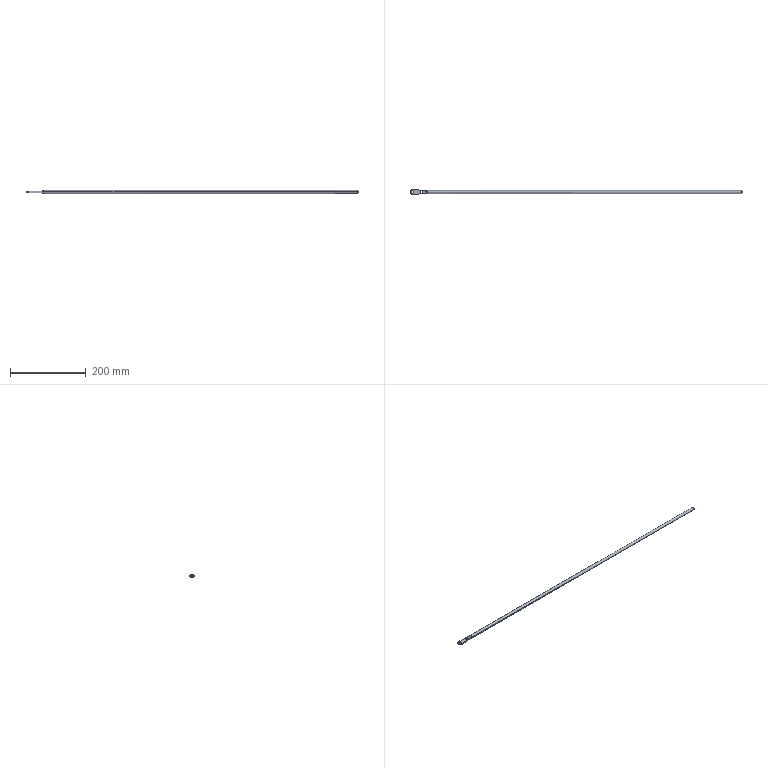Component | SolidWorks | RightRearDoorFrameAssembly-1_RearDoorLowerLockRod-1 | 1 solid | 20 faces | box 878.5 x 13 x 8 mm | volume 43100 mm3 | plane 11 | cylinder 7 | cone 2 | commonest cylinder face diameters 6.5 x4 8 x2 13 x1
build123d program:
from build123d import *

# Parameters (mm, degrees)
SKETCH1_R           = 4
BOSS_EXTRUDE1_DEPTH = 878.5
CUT_EXTRUDE1_DEPTH  = 5
SKETCH3_W           = 42
SKETCH3_H           = 2.024
CUT_EXTRUDE2_DEPTH  = 10
BOSS_EXTRUDE2_DEPTH = 3
CUT_EXTRUDE3_DEPTH  = 3
SKETCH6_R           = 3.25
CUT_EXTRUDE4_DEPTH  = 3
CHAMFER1_SIZE       = 1.5


with BuildPart() as part:
    # Sketch1 → Boss-Extrude1 (new body)
    with BuildSketch(Plane(origin=(0, 0, 0), x_dir=(0, 0, -1), z_dir=(1, 0, 0))):
        Circle(SKETCH1_R)
    extrude(amount=-BOSS_EXTRUDE1_DEPTH)

    # Sketch2 → Cut-Extrude1 (cut, symmetric)
    with BuildSketch(Plane.XY):
        Polygon((-42, 1.5), (-45.678, 4), (-42, 4), (0, 4), (0, 1.5), align=None)
        Polygon((-45.678, -4), (-42, -4), (0, -4), (0, -1.5), (-42, -1.5), align=None)
    extrude(amount=CUT_EXTRUDE1_DEPTH, both=True, mode=Mode.SUBTRACT)

    # Sketch3 → Cut-Extrude2 (cut)
    with BuildSketch(Plane(origin=(0, 1.5, 0), x_dir=(1, 0, 0), z_dir=(0, 1, 0))):
        with Locations((-21, 2.988)):
            Rectangle(SKETCH3_W, SKETCH3_H)
        with Locations((-21, -2.988)):
            Rectangle(SKETCH3_W, SKETCH3_H)
    extrude(amount=-CUT_EXTRUDE2_DEPTH, mode=Mode.SUBTRACT)

    # Sketch4 → Boss-Extrude2 (add)
    with BuildSketch(Plane(origin=(0, 1.5, 0), x_dir=(1, 0, 0), z_dir=(0, 1, 0))):
        with BuildLine():
            Line((-42, -4), (-42, 4))
            Line((-42, 4), (-7.386, 6.439))
            ThreePointArc((-7.386, 6.439), (0, 0), (-7.386, -6.439))
            Line((-7.386, -6.439), (-42, -4))
        make_face()
    extrude(amount=-BOSS_EXTRUDE2_DEPTH)

    # Sketch5 → Cut-Extrude3 (cut)
    with BuildSketch(Plane(origin=(0, 1.5, 0), x_dir=(1, 0, 0), z_dir=(0, 1, 0))):
        with BuildLine():
            Line((-0.8017, 3.127), (2.344, 3.127))
            Line((2.344, 3.127), (2.344, -3.404))
            Line((2.344, -3.404), (-0.9628, -3.404))
            ThreePointArc((-0.9628, -3.404), (-0.001977, -0.1603), (-0.8017, 3.127))
        make_face()
    extrude(amount=-CUT_EXTRUDE3_DEPTH, mode=Mode.SUBTRACT)

    # Sketch6 → Cut-Extrude4 (cut)
    with BuildSketch(Plane(origin=(0, 1.5, 0), x_dir=(1, 0, 0), z_dir=(0, 1, 0))):
        with Locations(Location((-6, 0, 0), (0, 0, 180))):
            Circle(SKETCH6_R)
        with Locations(Location((-31, 0, 0), (0, 0, 180))):
            Circle(SKETCH6_R)
    extrude(amount=-CUT_EXTRUDE4_DEPTH, mode=Mode.SUBTRACT)

    # Chamfer1
    chamfer1_edges = [part.edges().sort_by_distance(p)[0] for p in [
        (-878.5, 0, 4),
    ]]
    chamfer(chamfer1_edges, length=CHAMFER1_SIZE)


solid = part.part

# Placed as in the assembly
solid = solid.moved(Location((30.814, 303.707, -28.746), (-90, 0, 180)))
STEP:
#1=COLOUR_RGB('',0.7922,0.8196,0.9333);
#2=FILL_AREA_STYLE_COLOUR('',#1);
#3=FILL_AREA_STYLE('',(#2));
#4=SURFACE_STYLE_FILL_AREA(#3);
#5=SURFACE_SIDE_STYLE('',(#4));
#6=SURFACE_STYLE_USAGE(.BOTH.,#5);
#7=PRESENTATION_STYLE_ASSIGNMENT((#6));
#8=CARTESIAN_POINT('',(35.8,12.055,-1.132));
#9=VERTEX_POINT('',#8);
#10=CARTESIAN_POINT('',(35.8,11.859,-1.132));
#11=VERTEX_POINT('',#10);
#12=CARTESIAN_POINT('',(35.8,11.957,-1.132));
#13=DIRECTION('',(1.,-0.,0.));
#14=DIRECTION('',(0.,-1.,0.));
#15=AXIS2_PLACEMENT_3D('',#12,#13,#14);
#16=CIRCLE('',#15,0.09843);
#17=EDGE_CURVE('',#9,#11,#16,.T.);
#18=ORIENTED_EDGE('',*,*,#17,.F.);
#19=CARTESIAN_POINT('',(35.741,12.114,-1.132));
#20=VERTEX_POINT('',#19);
#21=CARTESIAN_POINT('',(35.741,12.114,-1.132));
#22=DIRECTION('',(-0.7071,0.7071,-0.));
#23=VECTOR('',#22,39.37);
#24=LINE('',#21,#23);
#25=EDGE_CURVE('',#9,#20,#24,.T.);
#26=ORIENTED_EDGE('',*,*,#25,.T.);
#27=CARTESIAN_POINT('',(35.741,11.799,-1.132));
#28=VERTEX_POINT('',#27);
#29=CARTESIAN_POINT('',(35.741,11.957,-1.132));
#30=DIRECTION('',(-1.,0.,-0.));
#31=DIRECTION('',(0.,-1.,0.));
#32=AXIS2_PLACEMENT_3D('',#29,#30,#31);
#33=CIRCLE('',#32,0.1575);
#34=EDGE_CURVE('',#28,#20,#33,.T.);
#35=ORIENTED_EDGE('',*,*,#34,.F.);
#36=CARTESIAN_POINT('',(35.741,11.799,-1.132));
#37=DIRECTION('',(-0.7071,-0.7071,-0.));
#38=VECTOR('',#37,39.37);
#39=LINE('',#36,#38);
#40=EDGE_CURVE('',#11,#28,#39,.T.);
#41=ORIENTED_EDGE('',*,*,#40,.F.);
#42=EDGE_LOOP('',(#18,#26,#35,#41));
#43=FACE_OUTER_BOUND('',#42,.T.);
#44=CARTESIAN_POINT('',(35.741,11.957,-1.132));
#45=DIRECTION('',(-1.,0.,-0.));
#46=DIRECTION('',(0.,-1.,0.));
#47=AXIS2_PLACEMENT_3D('',#44,#45,#46);
#48=CONICAL_SURFACE('',#47,0.1575,0.7854);
#49=ADVANCED_FACE('',(#43),#48,.T.);
#50=CARTESIAN_POINT('',(2.306,11.957,-1.191));
#51=VERTEX_POINT('',#50);
#52=CARTESIAN_POINT('',(2.562,11.957,-1.191));
#53=VERTEX_POINT('',#52);
#54=CARTESIAN_POINT('',(2.434,11.957,-1.191));
#55=DIRECTION('',(-0.,-0.,1.));
#56=DIRECTION('',(1.,0.,0.));
#57=AXIS2_PLACEMENT_3D('',#54,#55,#56);
#58=CIRCLE('',#57,0.128);
#59=EDGE_CURVE('',#51,#53,#58,.T.);
#60=ORIENTED_EDGE('',*,*,#59,.F.);
#61=CARTESIAN_POINT('',(2.306,11.957,-1.073));
#62=VERTEX_POINT('',#61);
#63=CARTESIAN_POINT('',(2.306,11.957,-1.191));
#64=DIRECTION('',(-0.,-0.,1.));
#65=VECTOR('',#64,39.37);
#66=LINE('',#63,#65);
#67=EDGE_CURVE('',#51,#62,#66,.T.);
#68=ORIENTED_EDGE('',*,*,#67,.T.);
#69=CARTESIAN_POINT('',(2.562,11.957,-1.073));
#70=VERTEX_POINT('',#69);
#71=CARTESIAN_POINT('',(2.434,11.957,-1.073));
#72=DIRECTION('',(-0.,-0.,1.));
#73=DIRECTION('',(1.,0.,0.));
#74=AXIS2_PLACEMENT_3D('',#71,#72,#73);
#75=CIRCLE('',#74,0.128);
#76=EDGE_CURVE('',#62,#70,#75,.T.);
#77=ORIENTED_EDGE('',*,*,#76,.T.);
#78=CARTESIAN_POINT('',(2.562,11.957,-1.191));
#79=DIRECTION('',(-0.,-0.,1.));
#80=VECTOR('',#79,39.37);
#81=LINE('',#78,#80);
#82=EDGE_CURVE('',#53,#70,#81,.T.);
#83=ORIENTED_EDGE('',*,*,#82,.F.);
#84=EDGE_LOOP('',(#60,#68,#77,#83));
#85=FACE_OUTER_BOUND('',#84,.T.);
#86=CARTESIAN_POINT('',(2.434,11.957,-1.191));
#87=DIRECTION('',(-0.,-0.,1.));
#88=DIRECTION('',(1.,0.,0.));
#89=AXIS2_PLACEMENT_3D('',#86,#87,#88);
#90=CYLINDRICAL_SURFACE('',#89,0.128);
#91=ADVANCED_FACE('',(#85),#90,.F.);
#92=CARTESIAN_POINT('',(1.321,11.957,-1.191));
#93=VERTEX_POINT('',#92);
#94=CARTESIAN_POINT('',(1.577,11.957,-1.191));
#95=VERTEX_POINT('',#94);
#96=CARTESIAN_POINT('',(1.449,11.957,-1.191));
#97=DIRECTION('',(-0.,-0.,1.));
#98=DIRECTION('',(1.,0.,0.));
#99=AXIS2_PLACEMENT_3D('',#96,#97,#98);
#100=CIRCLE('',#99,0.128);
#101=EDGE_CURVE('',#93,#95,#100,.T.);
#102=ORIENTED_EDGE('',*,*,#101,.F.);
#103=CARTESIAN_POINT('',(1.321,11.957,-1.073));
#104=VERTEX_POINT('',#103);
#105=CARTESIAN_POINT('',(1.321,11.957,-1.191));
#106=DIRECTION('',(-0.,-0.,1.));
#107=VECTOR('',#106,39.37);
#108=LINE('',#105,#107);
#109=EDGE_CURVE('',#93,#104,#108,.T.);
#110=ORIENTED_EDGE('',*,*,#109,.T.);
#111=CARTESIAN_POINT('',(1.577,11.957,-1.073));
#112=VERTEX_POINT('',#111);
#113=CARTESIAN_POINT('',(1.449,11.957,-1.073));
#114=DIRECTION('',(-0.,-0.,1.));
#115=DIRECTION('',(1.,0.,0.));
#116=AXIS2_PLACEMENT_3D('',#113,#114,#115);
#117=CIRCLE('',#116,0.128);
#118=EDGE_CURVE('',#104,#112,#117,.T.);
#119=ORIENTED_EDGE('',*,*,#118,.T.);
#120=CARTESIAN_POINT('',(1.577,11.957,-1.191));
#121=DIRECTION('',(-0.,-0.,1.));
#122=VECTOR('',#121,39.37);
#123=LINE('',#120,#122);
#124=EDGE_CURVE('',#95,#112,#123,.T.);
#125=ORIENTED_EDGE('',*,*,#124,.F.);
#126=EDGE_LOOP('',(#102,#110,#119,#125));
#127=FACE_OUTER_BOUND('',#126,.T.);
#128=CARTESIAN_POINT('',(1.449,11.957,-1.191));
#129=DIRECTION('',(-0.,-0.,1.));
#130=DIRECTION('',(1.,0.,0.));
#131=AXIS2_PLACEMENT_3D('',#128,#129,#130);
#132=CYLINDRICAL_SURFACE('',#131,0.128);
#133=ADVANCED_FACE('',(#127),#132,.F.);
#134=ORIENTED_EDGE('',*,*,#34,.T.);
#135=CARTESIAN_POINT('',(2.867,12.114,-1.132));
#136=VERTEX_POINT('',#135);
#137=CARTESIAN_POINT('',(35.8,12.114,-1.132));
#138=DIRECTION('',(-1.,0.,-0.));
#139=VECTOR('',#138,39.37);
#140=LINE('',#137,#139);
#141=EDGE_CURVE('',#20,#136,#140,.T.);
#142=ORIENTED_EDGE('',*,*,#141,.T.);
#143=CARTESIAN_POINT('',(2.867,12.103,-1.073));
#144=VERTEX_POINT('',#143);
#145=CARTESIAN_POINT('',(2.867,11.957,-1.132));
#146=DIRECTION('',(-1.,0.,-0.));
#147=DIRECTION('',(0.,-0.,-1.));
#148=AXIS2_PLACEMENT_3D('',#145,#146,#147);
#149=CIRCLE('',#148,0.1575);
#150=EDGE_CURVE('',#144,#136,#149,.T.);
#151=ORIENTED_EDGE('',*,*,#150,.F.);
#152=CARTESIAN_POINT('',(2.867,11.811,-1.073));
#153=VERTEX_POINT('',#152);
#154=CARTESIAN_POINT('',(2.867,11.811,-1.073));
#155=CARTESIAN_POINT('',(3.094,11.874,-0.918));
#156=CARTESIAN_POINT('',(3.094,12.04,-0.918));
#157=CARTESIAN_POINT('',(2.867,12.103,-1.073));
#158=(BOUNDED_CURVE()B_SPLINE_CURVE(3,(#154,#155,#156,#157),.UNSPECIFIED.,.F.,.F.)B_SPLINE_CURVE_WITH_KNOTS((4,4),(1.955,4.328),.UNSPECIFIED.)CURVE()GEOMETRIC_REPRESENTATION_ITEM()RATIONAL_B_SPLINE_CURVE((1.,0.5833,0.5833,1.))REPRESENTATION_ITEM(''));
#159=EDGE_CURVE('',#153,#144,#158,.T.);
#160=ORIENTED_EDGE('',*,*,#159,.F.);
#161=CARTESIAN_POINT('',(2.867,11.799,-1.132));
#162=VERTEX_POINT('',#161);
#163=CARTESIAN_POINT('',(2.867,11.957,-1.132));
#164=DIRECTION('',(-1.,0.,-0.));
#165=DIRECTION('',(0.,-0.,-1.));
#166=AXIS2_PLACEMENT_3D('',#163,#164,#165);
#167=CIRCLE('',#166,0.1575);
#168=EDGE_CURVE('',#162,#153,#167,.T.);
#169=ORIENTED_EDGE('',*,*,#168,.F.);
#170=CARTESIAN_POINT('',(35.8,11.799,-1.132));
#171=DIRECTION('',(-1.,0.,-0.));
#172=VECTOR('',#171,39.37);
#173=LINE('',#170,#172);
#174=EDGE_CURVE('',#28,#162,#173,.T.);
#175=ORIENTED_EDGE('',*,*,#174,.F.);
#176=EDGE_LOOP('',(#134,#142,#151,#160,#169,#175));
#177=FACE_OUTER_BOUND('',#176,.T.);
#178=CARTESIAN_POINT('',(35.8,11.957,-1.132));
#179=DIRECTION('',(-1.,0.,-0.));
#180=DIRECTION('',(0.,-1.,0.));
#181=AXIS2_PLACEMENT_3D('',#178,#179,#180);
#182=CYLINDRICAL_SURFACE('',#181,0.1575);
#183=ADVANCED_FACE('',(#177),#182,.T.);
#184=ORIENTED_EDGE('',*,*,#141,.F.);
#185=CARTESIAN_POINT('',(35.741,11.957,-1.132));
#186=DIRECTION('',(-1.,0.,-0.));
#187=DIRECTION('',(0.,-1.,0.));
#188=AXIS2_PLACEMENT_3D('',#185,#186,#187);
#189=CIRCLE('',#188,0.1575);
#190=EDGE_CURVE('',#20,#28,#189,.T.);
#191=ORIENTED_EDGE('',*,*,#190,.T.);
#192=ORIENTED_EDGE('',*,*,#174,.T.);
#193=CARTESIAN_POINT('',(2.867,11.811,-1.191));
#194=VERTEX_POINT('',#193);
#195=CARTESIAN_POINT('',(2.867,11.957,-1.132));
#196=DIRECTION('',(-1.,0.,-0.));
#197=DIRECTION('',(0.,-0.,-1.));
#198=AXIS2_PLACEMENT_3D('',#195,#196,#197);
#199=CIRCLE('',#198,0.1575);
#200=EDGE_CURVE('',#194,#162,#199,.T.);
#201=ORIENTED_EDGE('',*,*,#200,.F.);
#202=CARTESIAN_POINT('',(2.867,12.103,-1.191));
#203=VERTEX_POINT('',#202);
#204=CARTESIAN_POINT('',(2.867,12.103,-1.191));
#205=CARTESIAN_POINT('',(3.094,12.04,-1.345));
#206=CARTESIAN_POINT('',(3.094,11.874,-1.345));
#207=CARTESIAN_POINT('',(2.867,11.811,-1.191));
#208=(BOUNDED_CURVE()B_SPLINE_CURVE(3,(#204,#205,#206,#207),.UNSPECIFIED.,.F.,.F.)B_SPLINE_CURVE_WITH_KNOTS((4,4),(1.955,4.328),.UNSPECIFIED.)CURVE()GEOMETRIC_REPRESENTATION_ITEM()RATIONAL_B_SPLINE_CURVE((1.,0.5833,0.5833,1.))REPRESENTATION_ITEM(''));
#209=EDGE_CURVE('',#203,#194,#208,.T.);
#210=ORIENTED_EDGE('',*,*,#209,.F.);
#211=CARTESIAN_POINT('',(2.867,11.957,-1.132));
#212=DIRECTION('',(-1.,0.,-0.));
#213=DIRECTION('',(0.,0.,-1.));
#214=AXIS2_PLACEMENT_3D('',#211,#212,#213);
#215=CIRCLE('',#214,0.1575);
#216=EDGE_CURVE('',#136,#203,#215,.T.);
#217=ORIENTED_EDGE('',*,*,#216,.F.);
#218=EDGE_LOOP('',(#184,#191,#192,#201,#210,#217));
#219=FACE_OUTER_BOUND('',#218,.T.);
#220=CARTESIAN_POINT('',(35.8,11.957,-1.132));
#221=DIRECTION('',(-1.,0.,-0.));
#222=DIRECTION('',(0.,-1.,0.));
#223=AXIS2_PLACEMENT_3D('',#220,#221,#222);
#224=CYLINDRICAL_SURFACE('',#223,0.1575);
#225=ADVANCED_FACE('',(#219),#224,.T.);
#226=CARTESIAN_POINT('',(35.8,11.957,-1.132));
#227=DIRECTION('',(1.,-0.,0.));
#228=DIRECTION('',(0.,-1.,0.));
#229=AXIS2_PLACEMENT_3D('',#226,#227,#228);
#230=CIRCLE('',#229,0.09843);
#231=EDGE_CURVE('',#11,#9,#230,.T.);
#232=ORIENTED_EDGE('',*,*,#231,.T.);
#233=ORIENTED_EDGE('',*,*,#17,.T.);
#234=EDGE_LOOP('',(#232,#233));
#235=FACE_OUTER_BOUND('',#234,.T.);
#236=CARTESIAN_POINT('',(35.8,11.957,-1.132));
#237=DIRECTION('',(-1.,0.,-0.));
#238=DIRECTION('',(-0.,-1.,-0.));
#239=AXIS2_PLACEMENT_3D('',#236,#237,#238);
#240=PLANE('',#239);
#241=ADVANCED_FACE('',(#235),#240,.F.);
#242=CARTESIAN_POINT('',(2.434,11.957,-1.073));
#243=DIRECTION('',(-0.,-0.,1.));
#244=DIRECTION('',(1.,0.,0.));
#245=AXIS2_PLACEMENT_3D('',#242,#243,#244);
#246=CIRCLE('',#245,0.128);
#247=EDGE_CURVE('',#70,#62,#246,.T.);
#248=ORIENTED_EDGE('',*,*,#247,.F.);
#249=ORIENTED_EDGE('',*,*,#76,.F.);
#250=EDGE_LOOP('',(#248,#249));
#251=FACE_BOUND('',#250,.T.);
#252=CARTESIAN_POINT('',(1.449,11.957,-1.073));
#253=DIRECTION('',(-0.,-0.,1.));
#254=DIRECTION('',(1.,0.,0.));
#255=AXIS2_PLACEMENT_3D('',#252,#253,#254);
#256=CIRCLE('',#255,0.128);
#257=EDGE_CURVE('',#112,#104,#256,.T.);
#258=ORIENTED_EDGE('',*,*,#257,.F.);
#259=ORIENTED_EDGE('',*,*,#118,.F.);
#260=EDGE_LOOP('',(#258,#259));
#261=FACE_BOUND('',#260,.T.);
#262=CARTESIAN_POINT('',(2.867,12.114,-1.073));
#263=VERTEX_POINT('',#262);
#264=CARTESIAN_POINT('',(1.504,12.21,-1.073));
#265=VERTEX_POINT('',#264);
#266=CARTESIAN_POINT('',(2.867,12.114,-1.073));
#267=DIRECTION('',(-0.9975,0.0703,-0.));
#268=VECTOR('',#267,39.37);
#269=LINE('',#266,#268);
#270=EDGE_CURVE('',#263,#265,#269,.T.);
#271=ORIENTED_EDGE('',*,*,#270,.T.);
#272=CARTESIAN_POINT('',(1.504,11.703,-1.073));
#273=VERTEX_POINT('',#272);
#274=CARTESIAN_POINT('',(1.469,11.957,-1.073));
#275=DIRECTION('',(-0.,-0.,1.));
#276=DIRECTION('',(1.,0.,0.));
#277=AXIS2_PLACEMENT_3D('',#274,#275,#276);
#278=CIRCLE('',#277,0.2559);
#279=EDGE_CURVE('',#265,#273,#278,.T.);
#280=ORIENTED_EDGE('',*,*,#279,.T.);
#281=CARTESIAN_POINT('',(2.867,11.799,-1.073));
#282=VERTEX_POINT('',#281);
#283=CARTESIAN_POINT('',(2.867,11.799,-1.073));
#284=DIRECTION('',(0.9975,0.0703,0.));
#285=VECTOR('',#284,39.37);
#286=LINE('',#283,#285);
#287=EDGE_CURVE('',#273,#282,#286,.T.);
#288=ORIENTED_EDGE('',*,*,#287,.T.);
#289=CARTESIAN_POINT('',(2.867,12.114,-1.073));
#290=DIRECTION('',(0.,1.,0.));
#291=VECTOR('',#290,39.37);
#292=LINE('',#289,#291);
#293=EDGE_CURVE('',#282,#153,#292,.T.);
#294=ORIENTED_EDGE('',*,*,#293,.T.);
#295=CARTESIAN_POINT('',(2.867,11.76,-1.073));
#296=DIRECTION('',(0.,1.,0.));
#297=VECTOR('',#296,39.37);
#298=LINE('',#295,#297);
#299=EDGE_CURVE('',#153,#144,#298,.T.);
#300=ORIENTED_EDGE('',*,*,#299,.T.);
#301=CARTESIAN_POINT('',(2.867,12.114,-1.073));
#302=DIRECTION('',(0.,1.,0.));
#303=VECTOR('',#302,39.37);
#304=LINE('',#301,#303);
#305=EDGE_CURVE('',#144,#263,#304,.T.);
#306=ORIENTED_EDGE('',*,*,#305,.T.);
#307=EDGE_LOOP('',(#271,#280,#288,#294,#300,#306));
#308=FACE_OUTER_BOUND('',#307,.T.);
#309=CARTESIAN_POINT('',(1.213,11.76,-1.073));
#310=DIRECTION('',(0.,0.,-1.));
#311=DIRECTION('',(-1.,0.,-0.));
#312=AXIS2_PLACEMENT_3D('',#309,#310,#311);
#313=PLANE('',#312);
#314=ADVANCED_FACE('',(#251,#261,#308),#313,.F.);
#315=ORIENTED_EDGE('',*,*,#299,.F.);
#316=ORIENTED_EDGE('',*,*,#159,.T.);
#317=EDGE_LOOP('',(#315,#316));
#318=FACE_OUTER_BOUND('',#317,.T.);
#319=CARTESIAN_POINT('',(2.867,11.76,-1.073));
#320=DIRECTION('',(0.5621,-0.,-0.8271));
#321=DIRECTION('',(-0.8271,0.,-0.5621));
#322=AXIS2_PLACEMENT_3D('',#319,#320,#321);
#323=PLANE('',#322);
#324=ADVANCED_FACE('',(#318),#323,.F.);
#325=CARTESIAN_POINT('',(2.867,11.76,-1.191));
#326=DIRECTION('',(0.,1.,0.));
#327=VECTOR('',#326,39.37);
#328=LINE('',#325,#327);
#329=EDGE_CURVE('',#194,#203,#328,.T.);
#330=ORIENTED_EDGE('',*,*,#329,.T.);
#331=ORIENTED_EDGE('',*,*,#209,.T.);
#332=EDGE_LOOP('',(#330,#331));
#333=FACE_OUTER_BOUND('',#332,.T.);
#334=CARTESIAN_POINT('',(2.867,11.76,-1.191));
#335=DIRECTION('',(0.5621,-0.,0.8271));
#336=DIRECTION('',(0.8271,-0.,-0.5621));
#337=AXIS2_PLACEMENT_3D('',#334,#335,#336);
#338=PLANE('',#337);
#339=ADVANCED_FACE('',(#333),#338,.F.);
#340=CARTESIAN_POINT('',(2.434,11.957,-1.191));
#341=DIRECTION('',(-0.,-0.,1.));
#342=DIRECTION('',(1.,0.,0.));
#343=AXIS2_PLACEMENT_3D('',#340,#341,#342);
#344=CIRCLE('',#343,0.128);
#345=EDGE_CURVE('',#53,#51,#344,.T.);
#346=ORIENTED_EDGE('',*,*,#345,.T.);
#347=ORIENTED_EDGE('',*,*,#59,.T.);
#348=EDGE_LOOP('',(#346,#347));
#349=FACE_BOUND('',#348,.T.);
#350=CARTESIAN_POINT('',(1.449,11.957,-1.191));
#351=DIRECTION('',(-0.,-0.,1.));
#352=DIRECTION('',(1.,0.,0.));
#353=AXIS2_PLACEMENT_3D('',#350,#351,#352);
#354=CIRCLE('',#353,0.128);
#355=EDGE_CURVE('',#95,#93,#354,.T.);
#356=ORIENTED_EDGE('',*,*,#355,.T.);
#357=ORIENTED_EDGE('',*,*,#101,.T.);
#358=EDGE_LOOP('',(#356,#357));
#359=FACE_BOUND('',#358,.T.);
#360=CARTESIAN_POINT('',(1.504,12.21,-1.191));
#361=VERTEX_POINT('',#360);
#362=CARTESIAN_POINT('',(1.504,11.703,-1.191));
#363=VERTEX_POINT('',#362);
#364=CARTESIAN_POINT('',(1.469,11.957,-1.191));
#365=DIRECTION('',(-0.,-0.,1.));
#366=DIRECTION('',(1.,0.,0.));
#367=AXIS2_PLACEMENT_3D('',#364,#365,#366);
#368=CIRCLE('',#367,0.2559);
#369=EDGE_CURVE('',#361,#363,#368,.T.);
#370=ORIENTED_EDGE('',*,*,#369,.F.);
#371=CARTESIAN_POINT('',(2.867,12.114,-1.191));
#372=VERTEX_POINT('',#371);
#373=CARTESIAN_POINT('',(2.867,12.114,-1.191));
#374=DIRECTION('',(-0.9975,0.0703,-0.));
#375=VECTOR('',#374,39.37);
#376=LINE('',#373,#375);
#377=EDGE_CURVE('',#372,#361,#376,.T.);
#378=ORIENTED_EDGE('',*,*,#377,.F.);
#379=CARTESIAN_POINT('',(2.867,12.114,-1.191));
#380=DIRECTION('',(0.,1.,0.));
#381=VECTOR('',#380,39.37);
#382=LINE('',#379,#381);
#383=EDGE_CURVE('',#203,#372,#382,.T.);
#384=ORIENTED_EDGE('',*,*,#383,.F.);
#385=ORIENTED_EDGE('',*,*,#329,.F.);
#386=CARTESIAN_POINT('',(2.867,11.799,-1.191));
#387=VERTEX_POINT('',#386);
#388=CARTESIAN_POINT('',(2.867,12.114,-1.191));
#389=DIRECTION('',(0.,1.,0.));
#390=VECTOR('',#389,39.37);
#391=LINE('',#388,#390);
#392=EDGE_CURVE('',#387,#194,#391,.T.);
#393=ORIENTED_EDGE('',*,*,#392,.F.);
#394=CARTESIAN_POINT('',(2.867,11.799,-1.191));
#395=DIRECTION('',(0.9975,0.0703,0.));
#396=VECTOR('',#395,39.37);
#397=LINE('',#394,#396);
#398=EDGE_CURVE('',#363,#387,#397,.T.);
#399=ORIENTED_EDGE('',*,*,#398,.F.);
#400=EDGE_LOOP('',(#370,#378,#384,#385,#393,#399));
#401=FACE_OUTER_BOUND('',#400,.T.);
#402=CARTESIAN_POINT('',(1.213,11.76,-1.191));
#403=DIRECTION('',(-0.,-0.,1.));
#404=DIRECTION('',(1.,-0.,0.));
#405=AXIS2_PLACEMENT_3D('',#402,#403,#404);
#406=PLANE('',#405);
#407=ADVANCED_FACE('',(#349,#359,#401),#406,.F.);
#408=ORIENTED_EDGE('',*,*,#270,.F.);
#409=CARTESIAN_POINT('',(2.867,12.114,-1.191));
#410=DIRECTION('',(-0.,-0.,1.));
#411=VECTOR('',#410,39.37);
#412=LINE('',#409,#411);
#413=EDGE_CURVE('',#136,#263,#412,.T.);
#414=ORIENTED_EDGE('',*,*,#413,.F.);
#415=CARTESIAN_POINT('',(2.867,12.114,-1.191));
#416=DIRECTION('',(-0.,-0.,1.));
#417=VECTOR('',#416,39.37);
#418=LINE('',#415,#417);
#419=EDGE_CURVE('',#372,#136,#418,.T.);
#420=ORIENTED_EDGE('',*,*,#419,.F.);
#421=ORIENTED_EDGE('',*,*,#377,.T.);
#422=CARTESIAN_POINT('',(1.504,12.21,-1.191));
#423=DIRECTION('',(-0.,-0.,1.));
#424=VECTOR('',#423,39.37);
#425=LINE('',#422,#424);
#426=EDGE_CURVE('',#361,#265,#425,.T.);
#427=ORIENTED_EDGE('',*,*,#426,.T.);
#428=EDGE_LOOP('',(#408,#414,#420,#421,#427));
#429=FACE_OUTER_BOUND('',#428,.T.);
#430=CARTESIAN_POINT('',(2.867,12.114,-1.191));
#431=DIRECTION('',(0.0703,0.9975,0.));
#432=DIRECTION('',(-0.9975,0.0703,-0.));
#433=AXIS2_PLACEMENT_3D('',#430,#431,#432);
#434=PLANE('',#433);
#435=ADVANCED_FACE('',(#429),#434,.T.);
#436=ORIENTED_EDGE('',*,*,#419,.T.);
#437=ORIENTED_EDGE('',*,*,#216,.T.);
#438=ORIENTED_EDGE('',*,*,#383,.T.);
#439=EDGE_LOOP('',(#436,#437,#438));
#440=FACE_OUTER_BOUND('',#439,.T.);
#441=CARTESIAN_POINT('',(2.867,12.114,-1.191));
#442=DIRECTION('',(1.,-0.,0.));
#443=DIRECTION('',(0.,0.,-1.));
#444=AXIS2_PLACEMENT_3D('',#441,#442,#443);
#445=PLANE('',#444);
#446=ADVANCED_FACE('',(#440),#445,.T.);
#447=ORIENTED_EDGE('',*,*,#305,.F.);
#448=ORIENTED_EDGE('',*,*,#150,.T.);
#449=ORIENTED_EDGE('',*,*,#413,.T.);
#450=EDGE_LOOP('',(#447,#448,#449));
#451=FACE_OUTER_BOUND('',#450,.T.);
#452=CARTESIAN_POINT('',(2.867,12.114,-1.191));
#453=DIRECTION('',(1.,-0.,0.));
#454=DIRECTION('',(0.,0.,-1.));
#455=AXIS2_PLACEMENT_3D('',#452,#453,#454);
#456=PLANE('',#455);
#457=ADVANCED_FACE('',(#451),#456,.T.);
#458=ORIENTED_EDGE('',*,*,#392,.T.);
#459=ORIENTED_EDGE('',*,*,#200,.T.);
#460=CARTESIAN_POINT('',(2.867,11.799,-1.191));
#461=DIRECTION('',(-0.,-0.,1.));
#462=VECTOR('',#461,39.37);
#463=LINE('',#460,#462);
#464=EDGE_CURVE('',#387,#162,#463,.T.);
#465=ORIENTED_EDGE('',*,*,#464,.F.);
#466=EDGE_LOOP('',(#458,#459,#465));
#467=FACE_OUTER_BOUND('',#466,.T.);
#468=CARTESIAN_POINT('',(2.867,12.114,-1.191));
#469=DIRECTION('',(1.,-0.,0.));
#470=DIRECTION('',(0.,0.,-1.));
#471=AXIS2_PLACEMENT_3D('',#468,#469,#470);
#472=PLANE('',#471);
#473=ADVANCED_FACE('',(#467),#472,.T.);
#474=CARTESIAN_POINT('',(2.867,11.799,-1.191));
#475=DIRECTION('',(-0.,-0.,1.));
#476=VECTOR('',#475,39.37);
#477=LINE('',#474,#476);
#478=EDGE_CURVE('',#162,#282,#477,.T.);
#479=ORIENTED_EDGE('',*,*,#478,.F.);
#480=ORIENTED_EDGE('',*,*,#168,.T.);
#481=ORIENTED_EDGE('',*,*,#293,.F.);
#482=EDGE_LOOP('',(#479,#480,#481));
#483=FACE_OUTER_BOUND('',#482,.T.);
#484=CARTESIAN_POINT('',(2.867,12.114,-1.191));
#485=DIRECTION('',(1.,-0.,0.));
#486=DIRECTION('',(0.,0.,-1.));
#487=AXIS2_PLACEMENT_3D('',#484,#485,#486);
#488=PLANE('',#487);
#489=ADVANCED_FACE('',(#483),#488,.T.);
#490=CARTESIAN_POINT('',(1.504,11.703,-1.191));
#491=DIRECTION('',(-0.,-0.,1.));
#492=VECTOR('',#491,39.37);
#493=LINE('',#490,#492);
#494=EDGE_CURVE('',#363,#273,#493,.T.);
#495=ORIENTED_EDGE('',*,*,#494,.T.);
#496=ORIENTED_EDGE('',*,*,#279,.F.);
#497=ORIENTED_EDGE('',*,*,#426,.F.);
#498=ORIENTED_EDGE('',*,*,#369,.T.);
#499=EDGE_LOOP('',(#495,#496,#497,#498));
#500=FACE_OUTER_BOUND('',#499,.T.);
#501=CARTESIAN_POINT('',(1.469,11.957,-1.191));
#502=DIRECTION('',(-0.,-0.,1.));
#503=DIRECTION('',(1.,0.,0.));
#504=AXIS2_PLACEMENT_3D('',#501,#502,#503);
#505=CYLINDRICAL_SURFACE('',#504,0.2559);
#506=ADVANCED_FACE('',(#500),#505,.T.);
#507=ORIENTED_EDGE('',*,*,#287,.F.);
#508=ORIENTED_EDGE('',*,*,#494,.F.);
#509=ORIENTED_EDGE('',*,*,#398,.T.);
#510=ORIENTED_EDGE('',*,*,#464,.T.);
#511=ORIENTED_EDGE('',*,*,#478,.T.);
#512=EDGE_LOOP('',(#507,#508,#509,#510,#511));
#513=FACE_OUTER_BOUND('',#512,.T.);
#514=CARTESIAN_POINT('',(2.867,11.799,-1.191));
#515=DIRECTION('',(0.0703,-0.9975,-0.));
#516=DIRECTION('',(0.9975,0.0703,0.));
#517=AXIS2_PLACEMENT_3D('',#514,#515,#516);
#518=PLANE('',#517);
#519=ADVANCED_FACE('',(#513),#518,.T.);
#520=ORIENTED_EDGE('',*,*,#109,.F.);
#521=ORIENTED_EDGE('',*,*,#355,.F.);
#522=ORIENTED_EDGE('',*,*,#124,.T.);
#523=ORIENTED_EDGE('',*,*,#257,.T.);
#524=EDGE_LOOP('',(#520,#521,#522,#523));
#525=FACE_OUTER_BOUND('',#524,.T.);
#526=CARTESIAN_POINT('',(1.449,11.957,-1.191));
#527=DIRECTION('',(-0.,-0.,1.));
#528=DIRECTION('',(1.,0.,0.));
#529=AXIS2_PLACEMENT_3D('',#526,#527,#528);
#530=CYLINDRICAL_SURFACE('',#529,0.128);
#531=ADVANCED_FACE('',(#525),#530,.F.);
#532=ORIENTED_EDGE('',*,*,#67,.F.);
#533=ORIENTED_EDGE('',*,*,#345,.F.);
#534=ORIENTED_EDGE('',*,*,#82,.T.);
#535=ORIENTED_EDGE('',*,*,#247,.T.);
#536=EDGE_LOOP('',(#532,#533,#534,#535));
#537=FACE_OUTER_BOUND('',#536,.T.);
#538=CARTESIAN_POINT('',(2.434,11.957,-1.191));
#539=DIRECTION('',(-0.,-0.,1.));
#540=DIRECTION('',(1.,0.,0.));
#541=AXIS2_PLACEMENT_3D('',#538,#539,#540);
#542=CYLINDRICAL_SURFACE('',#541,0.128);
#543=ADVANCED_FACE('',(#537),#542,.F.);
#544=ORIENTED_EDGE('',*,*,#25,.F.);
#545=ORIENTED_EDGE('',*,*,#231,.F.);
#546=ORIENTED_EDGE('',*,*,#40,.T.);
#547=ORIENTED_EDGE('',*,*,#190,.F.);
#548=EDGE_LOOP('',(#544,#545,#546,#547));
#549=FACE_OUTER_BOUND('',#548,.T.);
#550=CARTESIAN_POINT('',(35.741,11.957,-1.132));
#551=DIRECTION('',(-1.,0.,-0.));
#552=DIRECTION('',(0.,-1.,0.));
#553=AXIS2_PLACEMENT_3D('',#550,#551,#552);
#554=CONICAL_SURFACE('',#553,0.1575,0.7854);
#555=ADVANCED_FACE('',(#549),#554,.T.);
#556=CLOSED_SHELL('',(#49,#91,#133,#183,#225,#241,#314,#324,#339,#407,#435,#446,#457,#473,#489,#506,#519,#531,#543,#555));
#557=MANIFOLD_SOLID_BREP('',#556);
#558=STYLED_ITEM('',(#7),#557);
#559=(LENGTH_UNIT()NAMED_UNIT(*)SI_UNIT($,.METRE.));
#560=LENGTH_MEASURE_WITH_UNIT(LENGTH_MEASURE(0.0254),#559);
#561=DIMENSIONAL_EXPONENTS(1.,0.,0.,0.,0.,0.,0.);
#562=(CONVERSION_BASED_UNIT('',#560)LENGTH_UNIT()NAMED_UNIT(#561));
#563=UNCERTAINTY_MEASURE_WITH_UNIT(LENGTH_MEASURE(0.00001),#562,'','');
#564=(NAMED_UNIT(*)PLANE_ANGLE_UNIT()SI_UNIT($,.RADIAN.));
#565=(NAMED_UNIT(*)SI_UNIT($,.STERADIAN.)SOLID_ANGLE_UNIT());
#566=(GEOMETRIC_REPRESENTATION_CONTEXT(3)GLOBAL_UNCERTAINTY_ASSIGNED_CONTEXT((#563))GLOBAL_UNIT_ASSIGNED_CONTEXT((#562,#564,#565))REPRESENTATION_CONTEXT('',''));
#567=MECHANICAL_DESIGN_GEOMETRIC_PRESENTATION_REPRESENTATION('',(#558),#566);
#568=CARTESIAN_POINT('',(0.,0.,0.));
#569=DIRECTION('',(0.,0.,1.));
#570=DIRECTION('',(1.,0.,0.));
#571=AXIS2_PLACEMENT_3D('',#568,#569,#570);
#572=(LENGTH_UNIT()NAMED_UNIT(*)SI_UNIT($,.METRE.));
#573=LENGTH_MEASURE_WITH_UNIT(LENGTH_MEASURE(0.0254),#572);
#574=DIMENSIONAL_EXPONENTS(1.,0.,0.,0.,0.,0.,0.);
#575=(CONVERSION_BASED_UNIT('',#573)LENGTH_UNIT()NAMED_UNIT(#574));
#576=UNCERTAINTY_MEASURE_WITH_UNIT(LENGTH_MEASURE(0.00001),#575,'','');
#577=(NAMED_UNIT(*)PLANE_ANGLE_UNIT()SI_UNIT($,.RADIAN.));
#578=(NAMED_UNIT(*)SI_UNIT($,.STERADIAN.)SOLID_ANGLE_UNIT());
#579=(GEOMETRIC_REPRESENTATION_CONTEXT(3)GLOBAL_UNCERTAINTY_ASSIGNED_CONTEXT((#576))GLOBAL_UNIT_ASSIGNED_CONTEXT((#575,#577,#578))REPRESENTATION_CONTEXT('',''));
#580=ADVANCED_BREP_SHAPE_REPRESENTATION('',(#557,#571),#579);
#581=PRESENTATION_LAYER_ASSIGNMENT('','',(#558));